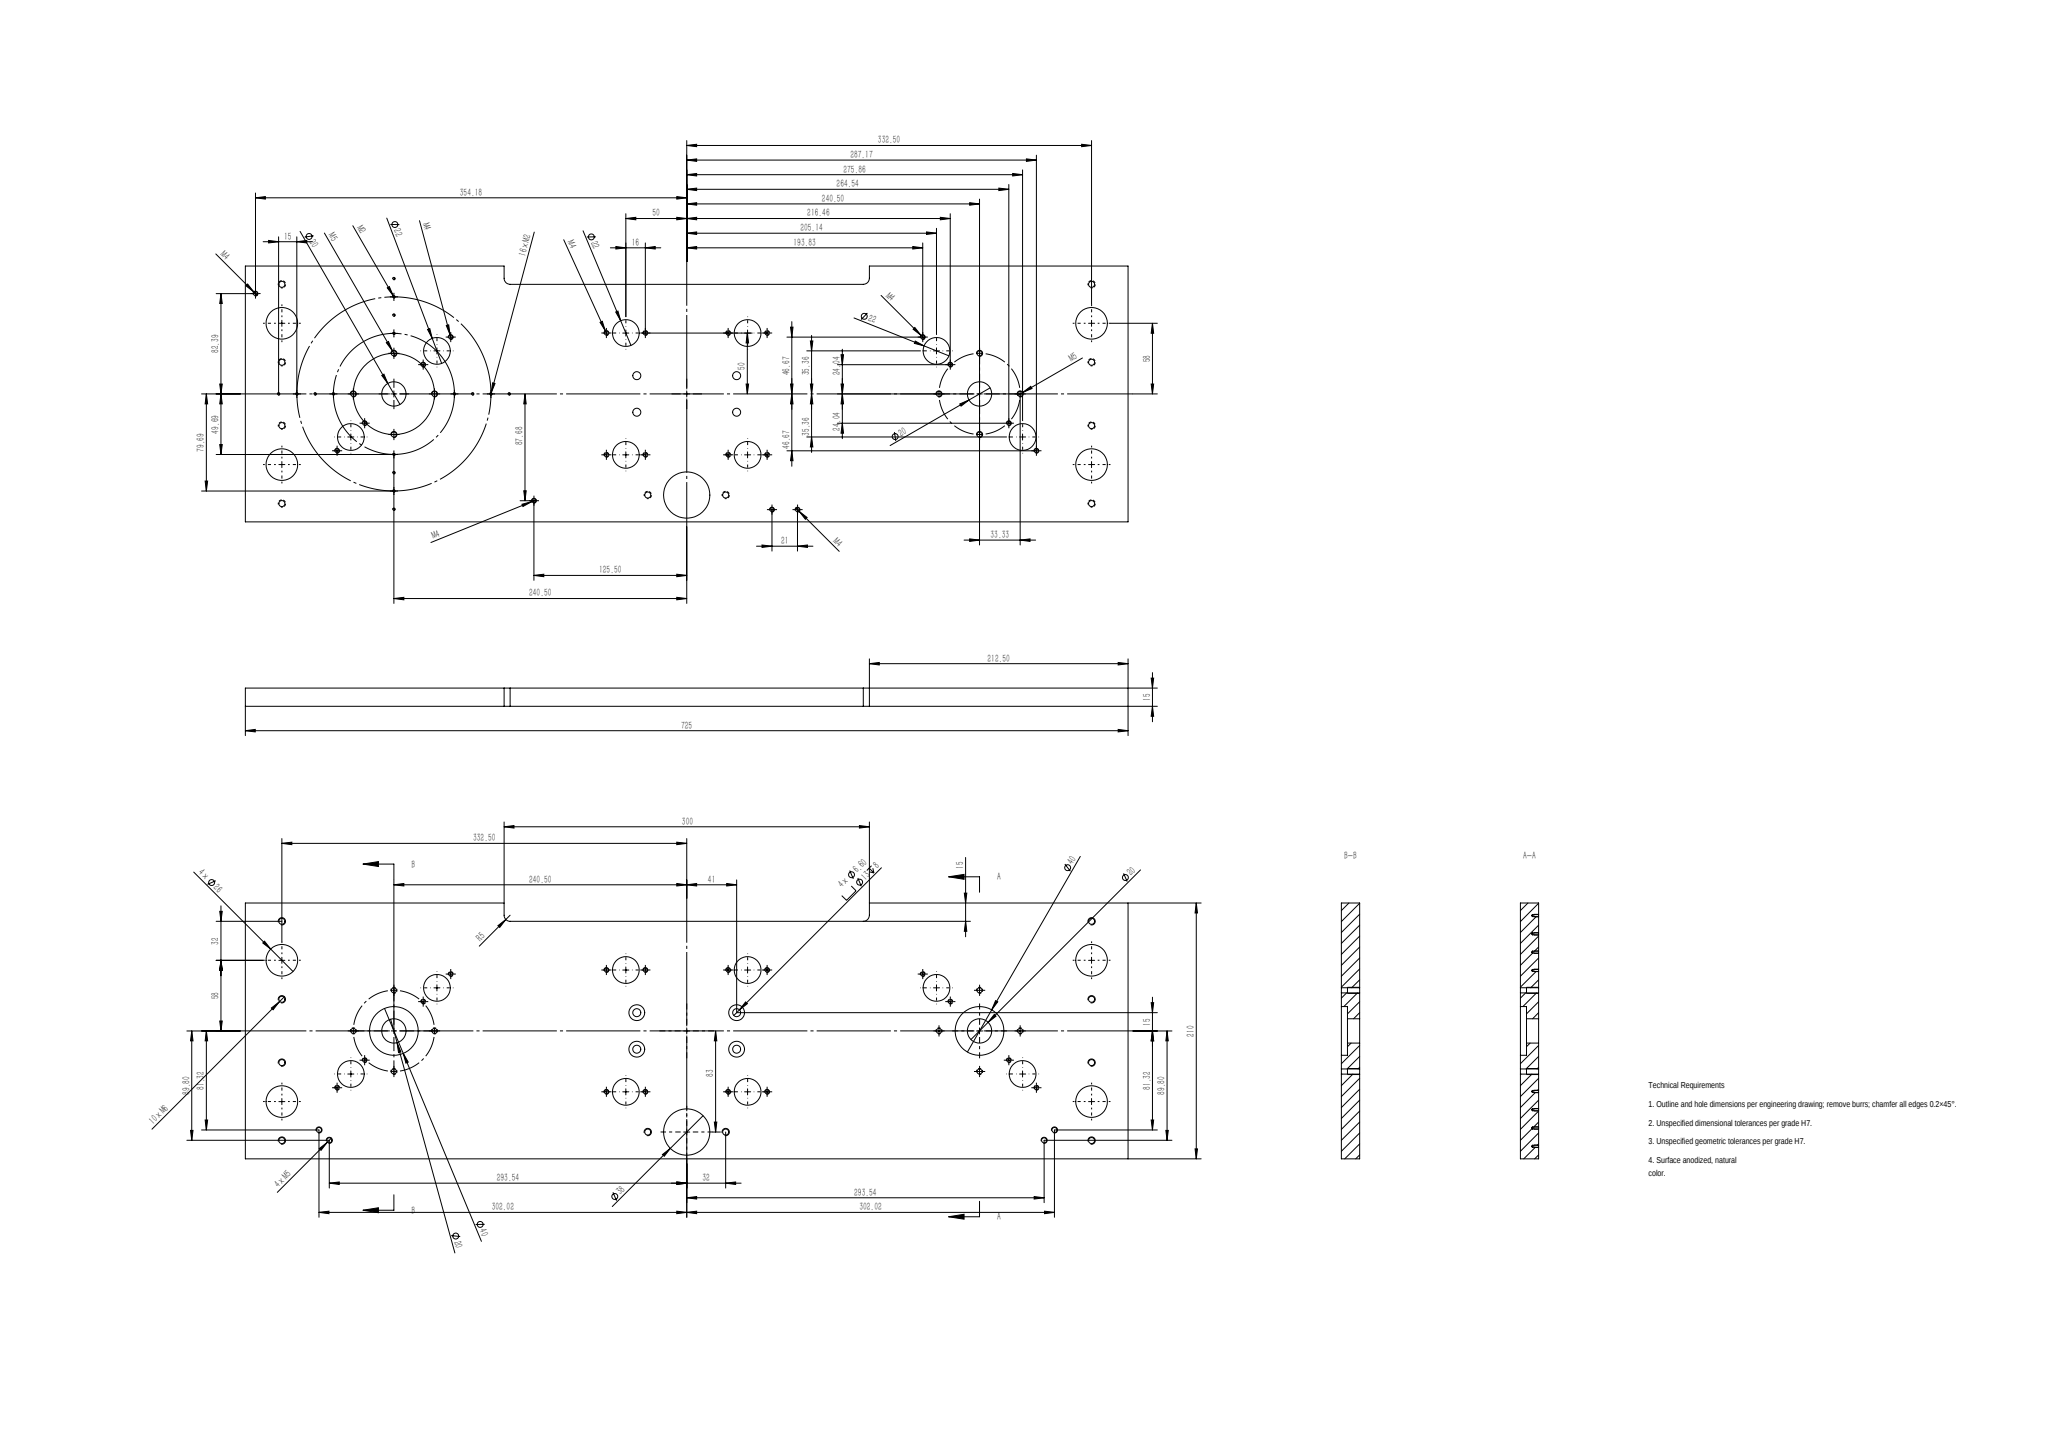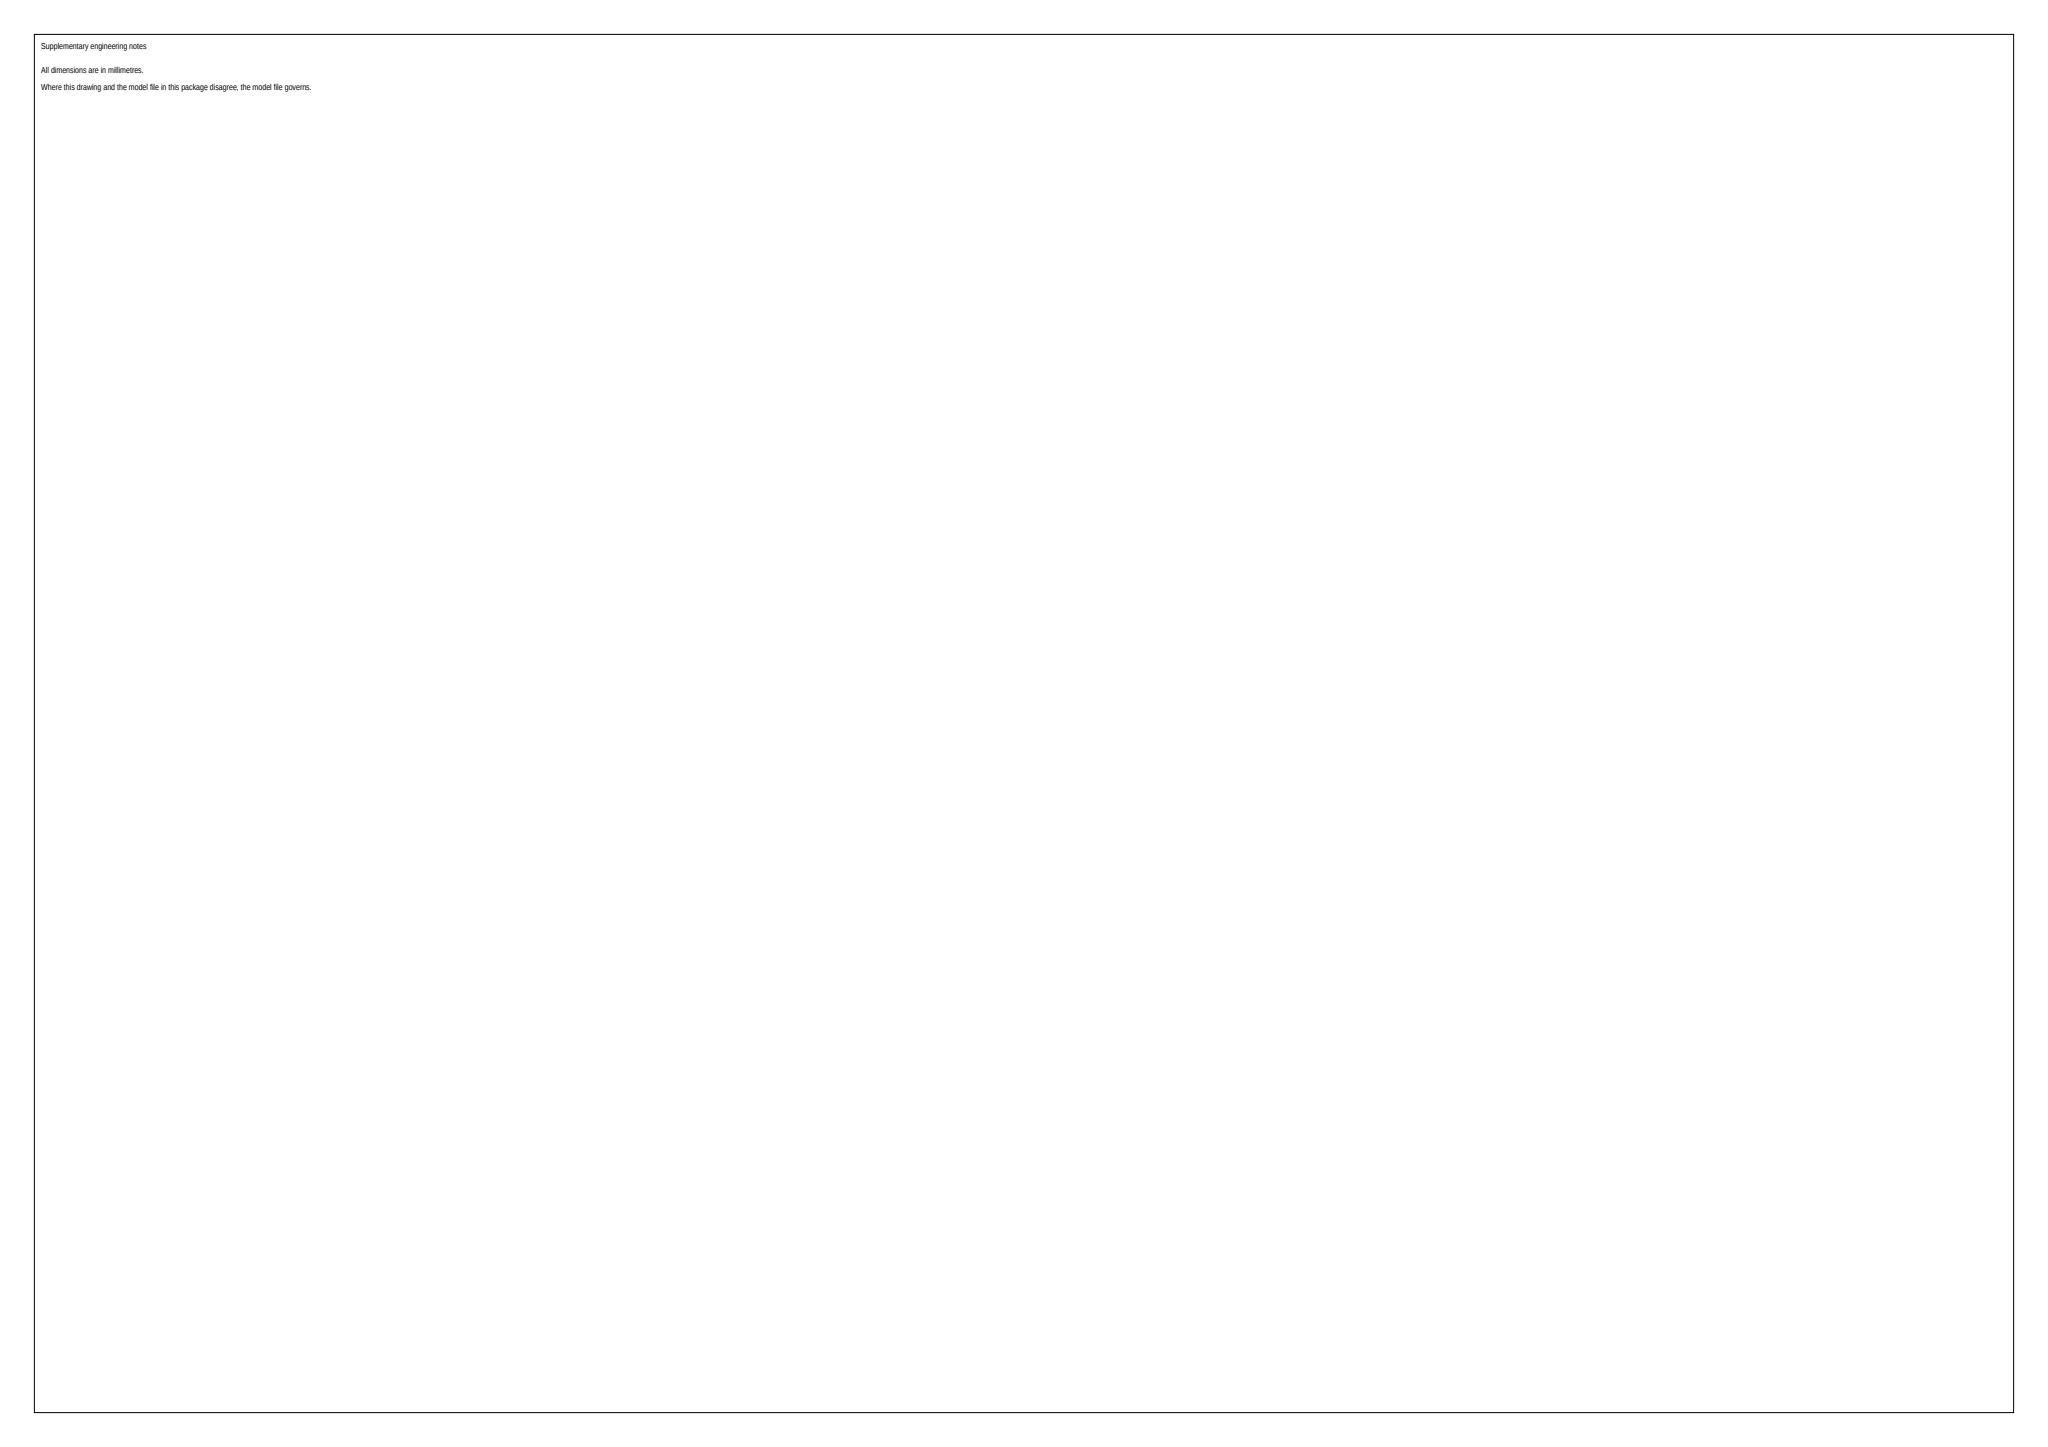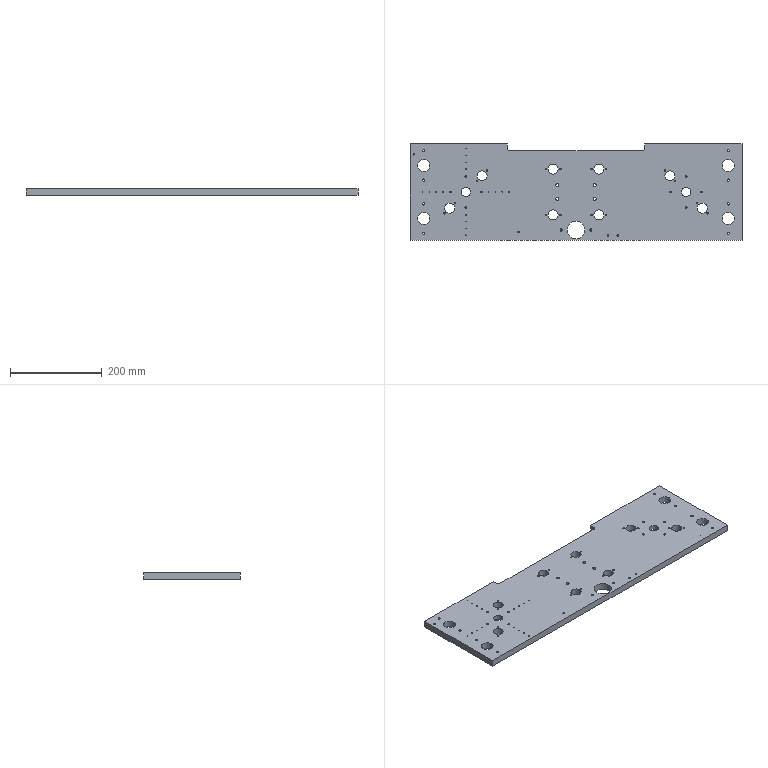Part | SolidWorks | mm | 1 solid | 232 faces | box 725 x 210 x 15 mm | volume 2089972 mm3 | cylinder 168 | cone 48 | plane 16 | commonest cylinder face diameters 3.3 x40 1.6 x32 4.2 x24 5 x20 22 x16 13 x8 6.6 x8 26 x8
build123d program:
from build123d import *

# Parameters (mm, degrees)
SKETCH1_W                                  = 725
SKETCH1_H                                  = 210
SKETCH1_R                                  = 13
SKETCH1_R_2                                = 19
BOSS_EXTRUDE1_DEPTH                        = 15
SKETCH2_R                                  = 11
SKETCH2_R_2                                = 10
CUT_EXTRUDE1_DEPTH                         = 15
M4_TAPPED_HOLE2_D                          = 3.3
M4_TAPPED_HOLE2_DEPTH                      = 15.1
M4_TAPPED_HOLE2_TIP                        = 0.9914
M2_TAPPED_HOLE1_AT_2_COUNT                 = 2
M2_TAPPED_HOLE1_AT_2_PITCH                 = 174.38
M2_TAPPED_HOLE1_AT_3_COUNT                 = 2
M2_TAPPED_HOLE1_AT_3_PITCH                 = 144.38
M2_TAPPED_HOLE1_AT_4_COUNT                 = 2
M2_TAPPED_HOLE1_AT_4_PITCH                 = 45
M2_TAPPED_HOLE1_AT_5_COUNT                 = 2
M2_TAPPED_HOLE1_AT_5_PITCH                 = 15
M2_TAPPED_HOLE1_AT_6_COUNT                 = 2
M2_TAPPED_HOLE1_AT_6_PITCH                 = 106.936
M2_TAPPED_HOLE1_AT_7_COUNT                 = 2
M2_TAPPED_HOLE1_AT_7_PITCH                 = 123.761
M2_TAPPED_HOLE1_AT_8_COUNT                 = 2
M2_TAPPED_HOLE1_AT_8_PITCH                 = 123.761
M2_TAPPED_HOLE1_AT_9_COUNT                 = 2
M2_TAPPED_HOLE1_AT_9_PITCH                 = 106.936
M2_TAPPED_HOLE1_AT_10_COUNT                = 2
M2_TAPPED_HOLE1_AT_10_PITCH                = 189.38
M2_TAPPED_HOLE1_AT_11_COUNT                = 2
M2_TAPPED_HOLE1_AT_11_PITCH                = 159.38
M2_TAPPED_HOLE1_AT_12_COUNT                = 2
M2_TAPPED_HOLE1_AT_12_PITCH                = 114.678
M2_TAPPED_HOLE1_AT_13_COUNT                = 2
M2_TAPPED_HOLE1_AT_13_PITCH                = 133.912
M2_TAPPED_HOLE1_AT_14_COUNT                = 2
M2_TAPPED_HOLE1_AT_14_PITCH                = 114.678
M2_TAPPED_HOLE1_AT_15_COUNT                = 2
M2_TAPPED_HOLE1_AT_15_PITCH                = 133.912
M2_TAPPED_HOLE1_AT_16_COUNT                = 2
M2_TAPPED_HOLE1_AT_16_PITCH                = 30
SKETCH26_R                                 = 20
CUT_EXTRUDE6_DEPTH                         = 5
CIRPATTERN3_COUNT                          = 4
M4_TAPPED_HOLE4_AT_2_COUNT                 = 2
M4_TAPPED_HOLE4_AT_2_PITCH                 = 132
M4_TAPPED_HOLE4_AT_3_COUNT                 = 2
M4_TAPPED_HOLE4_AT_3_PITCH                 = 100
M4_TAPPED_HOLE4_AT_4_COUNT                 = 2
M4_TAPPED_HOLE4_AT_4_PITCH                 = 32
M4_TAPPED_HOLE5_D                          = 3.3
M4_TAPPED_HOLE5_DEPTH                      = 10.1
M4_TAPPED_HOLE5_TIP                        = 0.9914
M4_TAPPED_HOLE6_D                          = 3.3
M4_TAPPED_HOLE6_DEPTH                      = 10.1
M4_TAPPED_HOLE6_TIP                        = 0.9914
M6_HEX_HEAD_BOLT_COUNTERBORE_1_D           = 6.6
M6_HEX_HEAD_BOLT_COUNTERBORE_1_CBORE_D     = 13
M6_HEX_HEAD_BOLT_COUNTERBORE_1_CBORE_DEPTH = 8
M6_TAPPED_HOLE1_D                          = 5
M6_TAPPED_HOLE1_DEPTH                      = 15
M6_TAPPED_HOLE1_TIP                        = 1.502
M5_TAPPED_HOLE5_D                          = 4.2
M5_TAPPED_HOLE5_DEPTH                      = 12.4
M5_TAPPED_HOLE5_TIP                        = 1.262
CUT_EXTRUDE7_DEPTH                         = 15


with BuildPart() as part:
    # Sketch1 → Boss-Extrude1 (new body)
    with BuildSketch(Plane.XY):
        Rectangle(SKETCH1_W, SKETCH1_H)
        with Locations((332.5, -58)):
            Circle(SKETCH1_R, mode=Mode.SUBTRACT)
        with Locations((332.5, 58)):
            Circle(SKETCH1_R, mode=Mode.SUBTRACT)
        with Locations((0, -83)):
            Circle(SKETCH1_R_2, mode=Mode.SUBTRACT)
        with Locations((-332.5, -58)):
            Circle(SKETCH1_R, mode=Mode.SUBTRACT)
        with Locations((-332.5, 58)):
            Circle(SKETCH1_R, mode=Mode.SUBTRACT)
    extrude(amount=BOSS_EXTRUDE1_DEPTH)

    # Sketch2 → Cut-Extrude1 (cut)
    with BuildSketch(Plane.XY.offset(15)):
        with Locations((-275.855, -35.355)):
            Circle(SKETCH2_R)
        with Locations((-205.145, 35.355)):
            Circle(SKETCH2_R)
        with Locations((-50, 50)):
            Circle(SKETCH2_R)
        with Locations((50, 50)):
            Circle(SKETCH2_R)
        with Locations((-50, -50)):
            Circle(SKETCH2_R)
        with Locations((50, -50)):
            Circle(SKETCH2_R)
        with Locations((-240.5, 0)):
            Circle(SKETCH2_R_2)
    cut_extrude1 = extrude(amount=-CUT_EXTRUDE1_DEPTH, mode=Mode.SUBTRACT)

    # Mirror1: Cut-Extrude1 across plane
    add(cut_extrude1.mirror(Plane(origin=(0, 0, 0), x_dir=(0, 0, 1), z_dir=(1, 0, 0))), mode=Mode.SUBTRACT)

    # M4 Tapped Hole2
    with Locations(Plane(origin=(0, 0, 0), x_dir=(-1, 0, 0), z_dir=(0, 0, -1))):
        with Locations((-66, -50), (66, 50), (34, 50), (-34, 50), (-66, 50), (66, -50), (34, -50), (-34, -50)):
            Hole(M4_TAPPED_HOLE2_D / 2, depth=M4_TAPPED_HOLE2_DEPTH)
            with Locations((0, 0, -(M4_TAPPED_HOLE2_DEPTH + M4_TAPPED_HOLE2_TIP / 2))):  # 118° drill point
                Cone(0, M4_TAPPED_HOLE2_D / 2, M4_TAPPED_HOLE2_TIP, mode=Mode.SUBTRACT)

    # Sketch23 → M2 Tapped Hole1 (revolve, cut)
    with BuildSketch(Plane(origin=(-145.81, 0, 15), x_dir=(0, -1, 0), z_dir=(1, 0, 0))):
        Polygon((0, 0), (0, 5.681), (0.8, 5.2), (0.8, 0), align=None)
    m2_tapped_hole1 = revolve(axis=Axis((-145.81, 0, 21.35), (0, 0, -1)), mode=Mode.SUBTRACT)

    # M2 Tapped Hole1 at 2: M2 Tapped Hole1 ×2
    with Locations(*[(-i * M2_TAPPED_HOLE1_AT_2_PITCH, 0, 0) for i in range(1, M2_TAPPED_HOLE1_AT_2_COUNT)]):
        add(m2_tapped_hole1, mode=Mode.SUBTRACT)

    # M2 Tapped Hole1 at 3: M2 Tapped Hole1 ×2
    with Locations(*[(-i * M2_TAPPED_HOLE1_AT_3_PITCH, 0, 0) for i in range(1, M2_TAPPED_HOLE1_AT_3_COUNT)]):
        add(m2_tapped_hole1, mode=Mode.SUBTRACT)

    # M2 Tapped Hole1 at 4: M2 Tapped Hole1 ×2
    with Locations(*[(-i * M2_TAPPED_HOLE1_AT_4_PITCH, 0, 0) for i in range(1, M2_TAPPED_HOLE1_AT_4_COUNT)]):
        add(m2_tapped_hole1, mode=Mode.SUBTRACT)

    # M2 Tapped Hole1 at 5: M2 Tapped Hole1 ×2
    with Locations(*[(-i * M2_TAPPED_HOLE1_AT_5_PITCH, 0, 0) for i in range(1, M2_TAPPED_HOLE1_AT_5_COUNT)]):
        add(m2_tapped_hole1, mode=Mode.SUBTRACT)

    # M2 Tapped Hole1 at 6: M2 Tapped Hole1 ×2
    with Locations(*[Vector(-0.8855, 0.4647, 0) * (i * M2_TAPPED_HOLE1_AT_6_PITCH) for i in range(1, M2_TAPPED_HOLE1_AT_6_COUNT)]):
        add(m2_tapped_hole1, mode=Mode.SUBTRACT)

    # M2 Tapped Hole1 at 7: M2 Tapped Hole1 ×2
    with Locations(*[Vector(-0.7651, 0.6439, 0) * (i * M2_TAPPED_HOLE1_AT_7_PITCH) for i in range(1, M2_TAPPED_HOLE1_AT_7_COUNT)]):
        add(m2_tapped_hole1, mode=Mode.SUBTRACT)

    # M2 Tapped Hole1 at 8: M2 Tapped Hole1 ×2
    with Locations(*[Vector(-0.7651, -0.6439, 0) * (i * M2_TAPPED_HOLE1_AT_8_PITCH) for i in range(1, M2_TAPPED_HOLE1_AT_8_COUNT)]):
        add(m2_tapped_hole1, mode=Mode.SUBTRACT)

    # M2 Tapped Hole1 at 9: M2 Tapped Hole1 ×2
    with Locations(*[Vector(-0.8855, -0.4647, 0) * (i * M2_TAPPED_HOLE1_AT_9_PITCH) for i in range(1, M2_TAPPED_HOLE1_AT_9_COUNT)]):
        add(m2_tapped_hole1, mode=Mode.SUBTRACT)

    # M2 Tapped Hole1 at 10: M2 Tapped Hole1 ×2
    with Locations(*[(-i * M2_TAPPED_HOLE1_AT_10_PITCH, 0, 0) for i in range(1, M2_TAPPED_HOLE1_AT_10_COUNT)]):
        add(m2_tapped_hole1, mode=Mode.SUBTRACT)

    # M2 Tapped Hole1 at 11: M2 Tapped Hole1 ×2
    with Locations(*[(-i * M2_TAPPED_HOLE1_AT_11_PITCH, 0, 0) for i in range(1, M2_TAPPED_HOLE1_AT_11_COUNT)]):
        add(m2_tapped_hole1, mode=Mode.SUBTRACT)

    # M2 Tapped Hole1 at 12: M2 Tapped Hole1 ×2
    with Locations(*[Vector(-0.8257, 0.5641, 0) * (i * M2_TAPPED_HOLE1_AT_12_PITCH) for i in range(1, M2_TAPPED_HOLE1_AT_12_COUNT)]):
        add(m2_tapped_hole1, mode=Mode.SUBTRACT)

    # M2 Tapped Hole1 at 13: M2 Tapped Hole1 ×2
    with Locations(*[Vector(-0.7071, 0.7071, 0) * (i * M2_TAPPED_HOLE1_AT_13_PITCH) for i in range(1, M2_TAPPED_HOLE1_AT_13_COUNT)]):
        add(m2_tapped_hole1, mode=Mode.SUBTRACT)

    # M2 Tapped Hole1 at 14: M2 Tapped Hole1 ×2
    with Locations(*[Vector(-0.8257, -0.5641, 0) * (i * M2_TAPPED_HOLE1_AT_14_PITCH) for i in range(1, M2_TAPPED_HOLE1_AT_14_COUNT)]):
        add(m2_tapped_hole1, mode=Mode.SUBTRACT)

    # M2 Tapped Hole1 at 15: M2 Tapped Hole1 ×2
    with Locations(*[Vector(-0.7071, -0.7071, 0) * (i * M2_TAPPED_HOLE1_AT_15_PITCH) for i in range(1, M2_TAPPED_HOLE1_AT_15_COUNT)]):
        add(m2_tapped_hole1, mode=Mode.SUBTRACT)

    # M2 Tapped Hole1 at 16: M2 Tapped Hole1 ×2
    with Locations(*[(-i * M2_TAPPED_HOLE1_AT_16_PITCH, 0, 0) for i in range(1, M2_TAPPED_HOLE1_AT_16_COUNT)]):
        add(m2_tapped_hole1, mode=Mode.SUBTRACT)

    # Sketch26 → Cut-Extrude6 (cut)
    with BuildSketch(Plane(origin=(0, 0, 0), x_dir=(-1, 0, 0), z_dir=(0, 0, -1))):
        with Locations((-240.5, 0)):
            Circle(SKETCH26_R)
        with Locations((240.5, 0)):
            Circle(SKETCH26_R)
    extrude(amount=-CUT_EXTRUDE6_DEPTH, mode=Mode.SUBTRACT)

    # Sketch29 → M5 Tapped Hole4 (revolve, cut)
    with BuildSketch(Plane(origin=(240.5, 33.33, 15), x_dir=(0, -1, 0), z_dir=(1, 0, 0))):
        Polygon((0, 0), (0, 16.262), (2.1, 15), (2.1, 0), align=None)
    m5_tapped_hole4 = revolve(axis=Axis((240.5, 33.33, 21.35), (0, 0, -1)), mode=Mode.SUBTRACT)

    # CirPattern3: M5 Tapped Hole4 ×4 about axis
    cirpattern3_axis = Axis((240.5, 0, 0), (0, 0, 1))
    for i in range(1, CIRPATTERN3_COUNT):
        add(m5_tapped_hole4.rotate(cirpattern3_axis, i * 360 / CIRPATTERN3_COUNT), mode=Mode.SUBTRACT)

    # Mirror6: M5 Tapped Hole4 across plane
    add(m5_tapped_hole4.mirror(Plane(origin=(0, 0, 0), x_dir=(0, 0, 1), z_dir=(1, 0, 0))), mode=Mode.SUBTRACT)

    # Mirror6 copy 1 sketch → Mirror6 copy 1 (revolve, cut)
    with BuildSketch(Plane(origin=(-207.17, 0, 15), x_dir=(-1, 0, 0), z_dir=(0, 1, 0))):
        Polygon((0, 0), (0, -16.262), (2.1, -15), (2.1, 0), align=None)
    revolve(axis=Axis((-207.17, 0, 21.35), (0, 0, 1)), mode=Mode.SUBTRACT)

    # Mirror6 copy 2 sketch → Mirror6 copy 2 (revolve, cut)
    with BuildSketch(Plane(origin=(-240.5, -33.33, 15), x_dir=(0, 1, 0), z_dir=(1, 0, 0))):
        Polygon((0, 0), (0, -16.262), (2.1, -15), (2.1, 0), align=None)
    revolve(axis=Axis((-240.5, -33.33, 21.35), (0, 0, 1)), mode=Mode.SUBTRACT)

    # Mirror6 copy 3 sketch → Mirror6 copy 3 (revolve, cut)
    with BuildSketch(Plane(origin=(-273.83, 0, 15), x_dir=(1, 0, 0), z_dir=(0, -1, 0))):
        Polygon((0, 0), (0, -16.262), (2.1, -15), (2.1, 0), align=None)
    revolve(axis=Axis((-273.83, 0, 21.35), (0, 0, 1)), mode=Mode.SUBTRACT)

    # Sketch31 → M4 Tapped Hole4 (revolve, cut)
    with BuildSketch(Plane(origin=(-193.831, 46.669, 15), x_dir=(0, -1, 0), z_dir=(1, 0, 0))):
        Polygon((0, 0), (0, 15.991), (1.65, 15), (1.65, 0), align=None)
    m4_tapped_hole4 = revolve(axis=Axis((-193.831, 46.669, 21.35), (0, 0, -1)), mode=Mode.SUBTRACT)

    # M4 Tapped Hole4 at 2: M4 Tapped Hole4 ×2
    with Locations(*[Vector(-0.7071, -0.7071, 0) * (i * M4_TAPPED_HOLE4_AT_2_PITCH) for i in range(1, M4_TAPPED_HOLE4_AT_2_COUNT)]):
        add(m4_tapped_hole4, mode=Mode.SUBTRACT)

    # M4 Tapped Hole4 at 3: M4 Tapped Hole4 ×2
    with Locations(*[Vector(-0.7071, -0.7071, 0) * (i * M4_TAPPED_HOLE4_AT_3_PITCH) for i in range(1, M4_TAPPED_HOLE4_AT_3_COUNT)]):
        add(m4_tapped_hole4, mode=Mode.SUBTRACT)

    # M4 Tapped Hole4 at 4: M4 Tapped Hole4 ×2
    with Locations(*[Vector(-0.7071, -0.7071, 0) * (i * M4_TAPPED_HOLE4_AT_4_PITCH) for i in range(1, M4_TAPPED_HOLE4_AT_4_COUNT)]):
        add(m4_tapped_hole4, mode=Mode.SUBTRACT)

    # Mirror8: M4 Tapped Hole4 across plane
    add(m4_tapped_hole4.mirror(Plane(origin=(0, 0, 0), x_dir=(0, 0, 1), z_dir=(1, 0, 0))), mode=Mode.SUBTRACT)

    # Mirror8 copy 1 sketch → Mirror8 copy 1 (revolve, cut)
    with BuildSketch(Plane(origin=(287.169, -46.669, 15), x_dir=(0, -1, 0), z_dir=(-1, 0, 0))):
        Polygon((0, 0), (0, -15.991), (1.65, -15), (1.65, 0), align=None)
    revolve(axis=Axis((287.169, -46.669, 21.35), (0, 0, 1)), mode=Mode.SUBTRACT)

    # Mirror8 copy 2 sketch → Mirror8 copy 2 (revolve, cut)
    with BuildSketch(Plane(origin=(264.542, -24.042, 15), x_dir=(0, -1, 0), z_dir=(-1, 0, 0))):
        Polygon((0, 0), (0, -15.991), (1.65, -15), (1.65, 0), align=None)
    revolve(axis=Axis((264.542, -24.042, 21.35), (0, 0, 1)), mode=Mode.SUBTRACT)

    # Mirror8 copy 3 sketch → Mirror8 copy 3 (revolve, cut)
    with BuildSketch(Plane(origin=(216.458, 24.042, 15), x_dir=(0, -1, 0), z_dir=(-1, 0, 0))):
        Polygon((0, 0), (0, -15.991), (1.65, -15), (1.65, 0), align=None)
    revolve(axis=Axis((216.458, 24.042, 21.35), (0, 0, 1)), mode=Mode.SUBTRACT)

    # M4 Tapped Hole5
    with Locations(Plane.XY.offset(15)):
        with Locations((-354.18, 82.39), (-125.5, -87.68)):
            Hole(M4_TAPPED_HOLE5_D / 2, depth=M4_TAPPED_HOLE5_DEPTH)
            with Locations((0, 0, -(M4_TAPPED_HOLE5_DEPTH + M4_TAPPED_HOLE5_TIP / 2))):  # 118° drill point
                Cone(0, M4_TAPPED_HOLE5_D / 2, M4_TAPPED_HOLE5_TIP, mode=Mode.SUBTRACT)

    # M4 Tapped Hole6
    with Locations(Plane.XY.offset(15)):
        with Locations((70, -95), (91, -95)):
            Hole(M4_TAPPED_HOLE6_D / 2, depth=M4_TAPPED_HOLE6_DEPTH)
            with Locations((0, 0, -(M4_TAPPED_HOLE6_DEPTH + M4_TAPPED_HOLE6_TIP / 2))):  # 118° drill point
                Cone(0, M4_TAPPED_HOLE6_D / 2, M4_TAPPED_HOLE6_TIP, mode=Mode.SUBTRACT)

    # M6 Hex Head Bolt Counterbore 1 (through all)
    with Locations(Plane(origin=(0, 0, 0), x_dir=(-1, 0, 0), z_dir=(0, 0, -1))):
        with Locations((-41, -15), (41, -15), (41, 15), (-41, 15)):
            CounterBoreHole(M6_HEX_HEAD_BOLT_COUNTERBORE_1_D / 2, M6_HEX_HEAD_BOLT_COUNTERBORE_1_CBORE_D / 2, M6_HEX_HEAD_BOLT_COUNTERBORE_1_CBORE_DEPTH)

    # M6 Tapped Hole1
    with Locations(Plane(origin=(0, 0, 0), x_dir=(-1, 0, 0), z_dir=(0, 0, -1))):
        with Locations((-332.5, 90), (-332.5, 26), (-32, -83), (32, -83), (332.5, 26), (332.5, 90), (332.5, -90), (332.5, -26), (-332.5, -26), (-332.5, -90)):
            Hole(M6_TAPPED_HOLE1_D / 2, depth=M6_TAPPED_HOLE1_DEPTH)
            with Locations((0, 0, -(M6_TAPPED_HOLE1_DEPTH + M6_TAPPED_HOLE1_TIP / 2))):  # 118° drill point
                Cone(0, M6_TAPPED_HOLE1_D / 2, M6_TAPPED_HOLE1_TIP, mode=Mode.SUBTRACT)

    # M5 Tapped Hole5
    with Locations(Plane(origin=(0, 0, 0), x_dir=(-1, 0, 0), z_dir=(0, 0, -1))):
        with Locations((302.023, -81.317), (-302.023, -81.317), (-293.537, -89.803), (293.537, -89.803)):
            Hole(M5_TAPPED_HOLE5_D / 2, depth=M5_TAPPED_HOLE5_DEPTH)
            with Locations((0, 0, -(M5_TAPPED_HOLE5_DEPTH + M5_TAPPED_HOLE5_TIP / 2))):  # 118° drill point
                Cone(0, M5_TAPPED_HOLE5_D / 2, M5_TAPPED_HOLE5_TIP, mode=Mode.SUBTRACT)

    # Sketch44 → Cut-Extrude7 (cut)
    with BuildSketch(Plane.XY.offset(15)):
        with BuildLine():
            Line((-150, 105), (150, 105))
            Line((150, 105), (150, 95))
            ThreePointArc((150, 95), (148.536, 91.464), (145, 90))
            Line((145, 90), (-145, 90))
            ThreePointArc((-145, 90), (-148.536, 91.464), (-150, 95))
            Line((-150, 95), (-150, 105))
        make_face()
    extrude(amount=-CUT_EXTRUDE7_DEPTH, mode=Mode.SUBTRACT)


solid = part.part